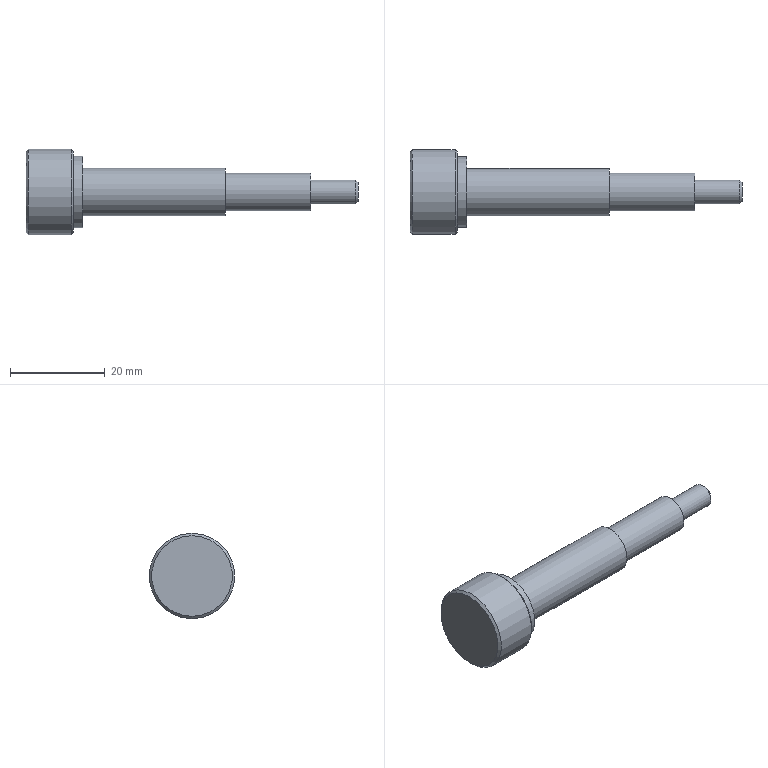Component | NX | CYLINDER_SHAFT | 1 solid | 14 faces | box 70 x 18 x 18 mm | volume 6340 mm3 | plane 6 | cylinder 5 | cone 3 | commonest cylinder face diameters 18 x1 15 x1 10 x1 8 x1 5 x1
STEP:
#1=CARTESIAN_POINT('',(0.,0.,0.));
#2=DIRECTION('',(0.,0.,1.));
#3=DIRECTION('',(1.,0.,0.));
#4=AXIS2_PLACEMENT_3D('',#1,#2,#3);
#5=CARTESIAN_POINT('',(-36.,0.,23.5));
#6=VERTEX_POINT('',#5);
#7=CARTESIAN_POINT('',(-36.,0.,32.));
#8=DIRECTION('',(1.,0.,0.));
#9=DIRECTION('',(0.,0.,-1.));
#10=AXIS2_PLACEMENT_3D('',#7,#8,#9);
#11=CIRCLE('',#10,8.5);
#12=CARTESIAN_POINT('',(-36.,0.,32.));
#13=DIRECTION('',(1.,0.,0.));
#14=DIRECTION('',(0.,0.,-1.));
#15=AXIS2_PLACEMENT_3D('',#12,#13,#14);
#16=PLANE('',#15);
#17=CARTESIAN_POINT('',(0.,0.));
#18=DIRECTION('',(1.,0.));
#19=AXIS2_PLACEMENT_2D('',#17,#18);
#20=CIRCLE('',#19,8.5);
#21=(GEOMETRIC_REPRESENTATION_CONTEXT(2)PARAMETRIC_REPRESENTATION_CONTEXT()REPRESENTATION_CONTEXT('',''));
#22=DEFINITIONAL_REPRESENTATION('',(#20),#21);
#23=PCURVE('',#16,#22);
#24=CARTESIAN_POINT('',(-36.5,0.,32.));
#25=DIRECTION('',(-1.,0.,0.));
#26=DIRECTION('',(0.,0.,1.));
#27=AXIS2_PLACEMENT_3D('',#24,#25,#26);
#28=CONICAL_SURFACE('',#27,9.,0.7854);
#29=CARTESIAN_POINT('',(9.425,-0.5));
#30=DIRECTION('',(-1.,0.));
#31=VECTOR('',#30,1.);
#32=LINE('',#29,#31);
#33=(GEOMETRIC_REPRESENTATION_CONTEXT(2)PARAMETRIC_REPRESENTATION_CONTEXT()REPRESENTATION_CONTEXT('',''));
#34=DEFINITIONAL_REPRESENTATION('',(#32),#33);
#35=PCURVE('',#28,#34);
#36=SURFACE_CURVE('',#11,(#23,#35),.PCURVE_S1.);
#37=EDGE_CURVE('',#6,#6,#36,.T.);
#38=ORIENTED_EDGE('',*,*,#37,.T.);
#39=EDGE_LOOP('',(#38));
#40=FACE_BOUND('',#39,.T.);
#41=CARTESIAN_POINT('',(-36.,0.,24.5));
#42=VERTEX_POINT('',#41);
#43=CARTESIAN_POINT('',(-36.,0.,32.));
#44=DIRECTION('',(1.,0.,0.));
#45=DIRECTION('',(0.,0.,-1.));
#46=AXIS2_PLACEMENT_3D('',#43,#44,#45);
#47=CIRCLE('',#46,7.5);
#48=CARTESIAN_POINT('',(0.,0.));
#49=DIRECTION('',(1.,0.));
#50=AXIS2_PLACEMENT_2D('',#48,#49);
#51=CIRCLE('',#50,7.5);
#52=(GEOMETRIC_REPRESENTATION_CONTEXT(2)PARAMETRIC_REPRESENTATION_CONTEXT()REPRESENTATION_CONTEXT('',''));
#53=DEFINITIONAL_REPRESENTATION('',(#51),#52);
#54=PCURVE('',#16,#53);
#55=CARTESIAN_POINT('',(-36.,0.,32.));
#56=DIRECTION('',(1.,0.,0.));
#57=DIRECTION('',(0.,0.,-1.));
#58=AXIS2_PLACEMENT_3D('',#55,#56,#57);
#59=CYLINDRICAL_SURFACE('',#58,7.5);
#60=CARTESIAN_POINT('',(0.,0.));
#61=DIRECTION('',(1.,0.));
#62=VECTOR('',#61,1.);
#63=LINE('',#60,#62);
#64=(GEOMETRIC_REPRESENTATION_CONTEXT(2)PARAMETRIC_REPRESENTATION_CONTEXT()REPRESENTATION_CONTEXT('',''));
#65=DEFINITIONAL_REPRESENTATION('',(#63),#64);
#66=PCURVE('',#59,#65);
#67=SURFACE_CURVE('',#47,(#54,#66),.PCURVE_S1.);
#68=EDGE_CURVE('',#42,#42,#67,.T.);
#69=ORIENTED_EDGE('',*,*,#68,.F.);
#70=EDGE_LOOP('',(#69));
#71=FACE_BOUND('',#70,.T.);
#72=ADVANCED_FACE('',(#40,#71),#16,.T.);
#73=CARTESIAN_POINT('',(-46.,0.,40.5));
#74=VERTEX_POINT('',#73);
#75=CARTESIAN_POINT('',(-46.,0.,32.));
#76=DIRECTION('',(-1.,0.,0.));
#77=DIRECTION('',(0.,0.,1.));
#78=AXIS2_PLACEMENT_3D('',#75,#76,#77);
#79=CIRCLE('',#78,8.5);
#80=CARTESIAN_POINT('',(-46.,0.,32.));
#81=DIRECTION('',(-1.,0.,0.));
#82=DIRECTION('',(0.,0.,1.));
#83=AXIS2_PLACEMENT_3D('',#80,#81,#82);
#84=PLANE('',#83);
#85=CARTESIAN_POINT('',(0.,0.));
#86=DIRECTION('',(1.,0.));
#87=AXIS2_PLACEMENT_2D('',#85,#86);
#88=CIRCLE('',#87,8.5);
#89=(GEOMETRIC_REPRESENTATION_CONTEXT(2)PARAMETRIC_REPRESENTATION_CONTEXT()REPRESENTATION_CONTEXT('',''));
#90=DEFINITIONAL_REPRESENTATION('',(#88),#89);
#91=PCURVE('',#84,#90);
#92=CARTESIAN_POINT('',(-45.5,0.,32.));
#93=DIRECTION('',(1.,0.,0.));
#94=DIRECTION('',(0.,0.,-1.));
#95=AXIS2_PLACEMENT_3D('',#92,#93,#94);
#96=CONICAL_SURFACE('',#95,9.,0.7854);
#97=CARTESIAN_POINT('',(9.425,-0.5));
#98=DIRECTION('',(-1.,0.));
#99=VECTOR('',#98,1.);
#100=LINE('',#97,#99);
#101=(GEOMETRIC_REPRESENTATION_CONTEXT(2)PARAMETRIC_REPRESENTATION_CONTEXT()REPRESENTATION_CONTEXT('',''));
#102=DEFINITIONAL_REPRESENTATION('',(#100),#101);
#103=PCURVE('',#96,#102);
#104=SURFACE_CURVE('',#79,(#91,#103),.PCURVE_S1.);
#105=EDGE_CURVE('',#74,#74,#104,.T.);
#106=ORIENTED_EDGE('',*,*,#105,.T.);
#107=EDGE_LOOP('',(#106));
#108=FACE_BOUND('',#107,.T.);
#109=ADVANCED_FACE('',(#108),#84,.T.);
#110=CARTESIAN_POINT('',(-45.5,0.,41.));
#111=VERTEX_POINT('',#110);
#112=CARTESIAN_POINT('',(-45.5,-0.,23.));
#113=VERTEX_POINT('',#112);
#114=CARTESIAN_POINT('',(-45.5,0.,32.));
#115=DIRECTION('',(1.,0.,0.));
#116=DIRECTION('',(0.,0.,1.));
#117=AXIS2_PLACEMENT_3D('',#114,#115,#116);
#118=CIRCLE('',#117,9.);
#119=CARTESIAN_POINT('',(-46.,0.,32.));
#120=DIRECTION('',(1.,0.,0.));
#121=DIRECTION('',(0.,0.,-1.));
#122=AXIS2_PLACEMENT_3D('',#119,#120,#121);
#123=CYLINDRICAL_SURFACE('',#122,9.);
#124=CARTESIAN_POINT('',(3.142,0.5));
#125=DIRECTION('',(1.,0.));
#126=VECTOR('',#125,1.);
#127=LINE('',#124,#126);
#128=(GEOMETRIC_REPRESENTATION_CONTEXT(2)PARAMETRIC_REPRESENTATION_CONTEXT()REPRESENTATION_CONTEXT('',''));
#129=DEFINITIONAL_REPRESENTATION('',(#127),#128);
#130=PCURVE('',#123,#129);
#131=CARTESIAN_POINT('',(3.142,0.));
#132=DIRECTION('',(1.,0.));
#133=VECTOR('',#132,1.);
#134=LINE('',#131,#133);
#135=(GEOMETRIC_REPRESENTATION_CONTEXT(2)PARAMETRIC_REPRESENTATION_CONTEXT()REPRESENTATION_CONTEXT('',''));
#136=DEFINITIONAL_REPRESENTATION('',(#134),#135);
#137=PCURVE('',#96,#136);
#138=SURFACE_CURVE('',#118,(#130,#137),.PCURVE_S1.);
#139=EDGE_CURVE('',#111,#113,#138,.T.);
#140=ORIENTED_EDGE('',*,*,#139,.T.);
#141=CARTESIAN_POINT('',(-36.5,0.,23.));
#142=VERTEX_POINT('',#141);
#143=CARTESIAN_POINT('',(-45.5,0.,23.));
#144=CARTESIAN_POINT('',(-36.5,0.,23.));
#145=B_SPLINE_CURVE_WITH_KNOTS('',1,(#143,#144),.UNSPECIFIED.,.F.,.F.,(2,2),(0.5,9.5),.PIECEWISE_BEZIER_KNOTS.);
#146=CARTESIAN_POINT('',(6.283,0.));
#147=DIRECTION('',(0.,1.));
#148=VECTOR('',#147,1.);
#149=LINE('',#146,#148);
#150=(GEOMETRIC_REPRESENTATION_CONTEXT(2)PARAMETRIC_REPRESENTATION_CONTEXT()REPRESENTATION_CONTEXT('',''));
#151=DEFINITIONAL_REPRESENTATION('',(#149),#150);
#152=PCURVE('',#123,#151);
#153=CARTESIAN_POINT('',(0.,0.));
#154=DIRECTION('',(0.,1.));
#155=VECTOR('',#154,1.);
#156=LINE('',#153,#155);
#157=(GEOMETRIC_REPRESENTATION_CONTEXT(2)PARAMETRIC_REPRESENTATION_CONTEXT()REPRESENTATION_CONTEXT('',''));
#158=DEFINITIONAL_REPRESENTATION('',(#156),#157);
#159=PCURVE('',#123,#158);
#160=SEAM_CURVE('',#145,(#152,#159),.PCURVE_S1.);
#161=EDGE_CURVE('',#113,#142,#160,.T.);
#162=ORIENTED_EDGE('',*,*,#161,.T.);
#163=CARTESIAN_POINT('',(-36.5,0.,32.));
#164=DIRECTION('',(-1.,0.,0.));
#165=DIRECTION('',(0.,0.,-1.));
#166=AXIS2_PLACEMENT_3D('',#163,#164,#165);
#167=CIRCLE('',#166,9.);
#168=CARTESIAN_POINT('',(6.283,9.5));
#169=DIRECTION('',(-1.,0.));
#170=VECTOR('',#169,1.);
#171=LINE('',#168,#170);
#172=(GEOMETRIC_REPRESENTATION_CONTEXT(2)PARAMETRIC_REPRESENTATION_CONTEXT()REPRESENTATION_CONTEXT('',''));
#173=DEFINITIONAL_REPRESENTATION('',(#171),#172);
#174=PCURVE('',#123,#173);
#175=CARTESIAN_POINT('',(3.142,0.));
#176=DIRECTION('',(1.,0.));
#177=VECTOR('',#176,1.);
#178=LINE('',#175,#177);
#179=(GEOMETRIC_REPRESENTATION_CONTEXT(2)PARAMETRIC_REPRESENTATION_CONTEXT()REPRESENTATION_CONTEXT('',''));
#180=DEFINITIONAL_REPRESENTATION('',(#178),#179);
#181=PCURVE('',#28,#180);
#182=SURFACE_CURVE('',#167,(#174,#181),.PCURVE_S1.);
#183=EDGE_CURVE('',#142,#142,#182,.T.);
#184=ORIENTED_EDGE('',*,*,#183,.T.);
#185=ORIENTED_EDGE('',*,*,#161,.F.);
#186=CARTESIAN_POINT('',(-45.5,0.,32.));
#187=DIRECTION('',(1.,0.,0.));
#188=DIRECTION('',(0.,0.,1.));
#189=AXIS2_PLACEMENT_3D('',#186,#187,#188);
#190=CIRCLE('',#189,9.);
#191=CARTESIAN_POINT('',(-3.142,0.5));
#192=DIRECTION('',(1.,0.));
#193=VECTOR('',#192,1.);
#194=LINE('',#191,#193);
#195=(GEOMETRIC_REPRESENTATION_CONTEXT(2)PARAMETRIC_REPRESENTATION_CONTEXT()REPRESENTATION_CONTEXT('',''));
#196=DEFINITIONAL_REPRESENTATION('',(#194),#195);
#197=PCURVE('',#123,#196);
#198=CARTESIAN_POINT('',(3.142,0.));
#199=DIRECTION('',(1.,0.));
#200=VECTOR('',#199,1.);
#201=LINE('',#198,#200);
#202=(GEOMETRIC_REPRESENTATION_CONTEXT(2)PARAMETRIC_REPRESENTATION_CONTEXT()REPRESENTATION_CONTEXT('',''));
#203=DEFINITIONAL_REPRESENTATION('',(#201),#202);
#204=PCURVE('',#96,#203);
#205=SURFACE_CURVE('',#190,(#197,#204),.PCURVE_S1.);
#206=EDGE_CURVE('',#113,#111,#205,.T.);
#207=ORIENTED_EDGE('',*,*,#206,.T.);
#208=EDGE_LOOP('',(#140,#162,#184,#185,#207));
#209=FACE_BOUND('',#208,.T.);
#210=ADVANCED_FACE('',(#209),#123,.T.);
#211=CARTESIAN_POINT('',(-34.,0.,27.));
#212=VERTEX_POINT('',#211);
#213=CARTESIAN_POINT('',(-34.,0.,32.));
#214=DIRECTION('',(1.,0.,0.));
#215=DIRECTION('',(0.,0.,-1.));
#216=AXIS2_PLACEMENT_3D('',#213,#214,#215);
#217=CIRCLE('',#216,5.);
#218=CARTESIAN_POINT('',(-34.,0.,32.));
#219=DIRECTION('',(1.,0.,0.));
#220=DIRECTION('',(0.,0.,-1.));
#221=AXIS2_PLACEMENT_3D('',#218,#219,#220);
#222=PLANE('',#221);
#223=CARTESIAN_POINT('',(0.,0.));
#224=DIRECTION('',(1.,0.));
#225=AXIS2_PLACEMENT_2D('',#223,#224);
#226=CIRCLE('',#225,5.);
#227=(GEOMETRIC_REPRESENTATION_CONTEXT(2)PARAMETRIC_REPRESENTATION_CONTEXT()REPRESENTATION_CONTEXT('',''));
#228=DEFINITIONAL_REPRESENTATION('',(#226),#227);
#229=PCURVE('',#222,#228);
#230=CARTESIAN_POINT('',(-34.,0.,32.));
#231=DIRECTION('',(1.,0.,0.));
#232=DIRECTION('',(0.,0.,-1.));
#233=AXIS2_PLACEMENT_3D('',#230,#231,#232);
#234=CYLINDRICAL_SURFACE('',#233,5.);
#235=CARTESIAN_POINT('',(0.,0.));
#236=DIRECTION('',(1.,0.));
#237=VECTOR('',#236,1.);
#238=LINE('',#235,#237);
#239=(GEOMETRIC_REPRESENTATION_CONTEXT(2)PARAMETRIC_REPRESENTATION_CONTEXT()REPRESENTATION_CONTEXT('',''));
#240=DEFINITIONAL_REPRESENTATION('',(#238),#239);
#241=PCURVE('',#234,#240);
#242=SURFACE_CURVE('',#217,(#229,#241),.PCURVE_S1.);
#243=EDGE_CURVE('',#212,#212,#242,.T.);
#244=ORIENTED_EDGE('',*,*,#243,.F.);
#245=EDGE_LOOP('',(#244));
#246=FACE_BOUND('',#245,.T.);
#247=CARTESIAN_POINT('',(-34.,0.,24.5));
#248=VERTEX_POINT('',#247);
#249=CARTESIAN_POINT('',(-34.,0.,32.));
#250=DIRECTION('',(-1.,0.,0.));
#251=DIRECTION('',(0.,0.,-1.));
#252=AXIS2_PLACEMENT_3D('',#249,#250,#251);
#253=CIRCLE('',#252,7.5);
#254=CARTESIAN_POINT('',(7.5,0.));
#255=CARTESIAN_POINT('',(7.5,-12.99));
#256=CARTESIAN_POINT('',(-3.75,-6.495));
#257=CARTESIAN_POINT('',(-15.,-0.));
#258=CARTESIAN_POINT('',(-3.75,6.495));
#259=CARTESIAN_POINT('',(7.5,12.99));
#260=CARTESIAN_POINT('',(7.5,0.));
#261=(BOUNDED_CURVE()B_SPLINE_CURVE(2,(#254,#255,#256,#257,#258,#259,#260),.UNSPECIFIED.,.T.,.F.)B_SPLINE_CURVE_WITH_KNOTS((1,2,2,2,2,1),(-2.094,0.,2.094,4.189,6.283,8.378),.UNSPECIFIED.)CURVE()GEOMETRIC_REPRESENTATION_ITEM()RATIONAL_B_SPLINE_CURVE((1.,0.5,1.,0.5,1.,0.5,1.))REPRESENTATION_ITEM(''));
#262=(GEOMETRIC_REPRESENTATION_CONTEXT(2)PARAMETRIC_REPRESENTATION_CONTEXT()REPRESENTATION_CONTEXT('',''));
#263=DEFINITIONAL_REPRESENTATION('',(#261),#262);
#264=PCURVE('',#222,#263);
#265=CARTESIAN_POINT('',(6.283,2.));
#266=DIRECTION('',(-1.,0.));
#267=VECTOR('',#266,1.);
#268=LINE('',#265,#267);
#269=(GEOMETRIC_REPRESENTATION_CONTEXT(2)PARAMETRIC_REPRESENTATION_CONTEXT()REPRESENTATION_CONTEXT('',''));
#270=DEFINITIONAL_REPRESENTATION('',(#268),#269);
#271=PCURVE('',#59,#270);
#272=SURFACE_CURVE('',#253,(#264,#271),.PCURVE_S1.);
#273=EDGE_CURVE('',#248,#248,#272,.T.);
#274=ORIENTED_EDGE('',*,*,#273,.F.);
#275=EDGE_LOOP('',(#274));
#276=FACE_BOUND('',#275,.T.);
#277=ADVANCED_FACE('',(#246,#276),#222,.T.);
#278=ORIENTED_EDGE('',*,*,#273,.T.);
#279=CARTESIAN_POINT('',(-36.,-0.,24.5));
#280=CARTESIAN_POINT('',(-34.,-0.,24.5));
#281=B_SPLINE_CURVE_WITH_KNOTS('',1,(#279,#280),.UNSPECIFIED.,.F.,.F.,(2,2),(0.,2.),.PIECEWISE_BEZIER_KNOTS.);
#282=CARTESIAN_POINT('',(0.,0.));
#283=DIRECTION('',(0.,1.));
#284=VECTOR('',#283,1.);
#285=LINE('',#282,#284);
#286=(GEOMETRIC_REPRESENTATION_CONTEXT(2)PARAMETRIC_REPRESENTATION_CONTEXT()REPRESENTATION_CONTEXT('',''));
#287=DEFINITIONAL_REPRESENTATION('',(#285),#286);
#288=PCURVE('',#59,#287);
#289=CARTESIAN_POINT('',(6.283,0.));
#290=DIRECTION('',(0.,1.));
#291=VECTOR('',#290,1.);
#292=LINE('',#289,#291);
#293=(GEOMETRIC_REPRESENTATION_CONTEXT(2)PARAMETRIC_REPRESENTATION_CONTEXT()REPRESENTATION_CONTEXT('',''));
#294=DEFINITIONAL_REPRESENTATION('',(#292),#293);
#295=PCURVE('',#59,#294);
#296=SEAM_CURVE('',#281,(#288,#295),.PCURVE_S1.);
#297=EDGE_CURVE('',#42,#248,#296,.T.);
#298=ORIENTED_EDGE('',*,*,#297,.F.);
#299=ORIENTED_EDGE('',*,*,#68,.T.);
#300=ORIENTED_EDGE('',*,*,#297,.T.);
#301=EDGE_LOOP('',(#278,#298,#299,#300));
#302=FACE_BOUND('',#301,.T.);
#303=ADVANCED_FACE('',(#302),#59,.T.);
#304=CARTESIAN_POINT('',(-4.,0.,28.));
#305=VERTEX_POINT('',#304);
#306=CARTESIAN_POINT('',(-4.,0.,32.));
#307=DIRECTION('',(1.,0.,0.));
#308=DIRECTION('',(0.,0.,-1.));
#309=AXIS2_PLACEMENT_3D('',#306,#307,#308);
#310=CIRCLE('',#309,4.);
#311=CARTESIAN_POINT('',(-4.,0.,32.));
#312=DIRECTION('',(1.,0.,0.));
#313=DIRECTION('',(0.,0.,-1.));
#314=AXIS2_PLACEMENT_3D('',#311,#312,#313);
#315=PLANE('',#314);
#316=CARTESIAN_POINT('',(0.,0.));
#317=DIRECTION('',(1.,0.));
#318=AXIS2_PLACEMENT_2D('',#316,#317);
#319=CIRCLE('',#318,4.);
#320=(GEOMETRIC_REPRESENTATION_CONTEXT(2)PARAMETRIC_REPRESENTATION_CONTEXT()REPRESENTATION_CONTEXT('',''));
#321=DEFINITIONAL_REPRESENTATION('',(#319),#320);
#322=PCURVE('',#315,#321);
#323=CARTESIAN_POINT('',(-4.,0.,32.));
#324=DIRECTION('',(1.,0.,0.));
#325=DIRECTION('',(0.,0.,-1.));
#326=AXIS2_PLACEMENT_3D('',#323,#324,#325);
#327=CYLINDRICAL_SURFACE('',#326,4.);
#328=CARTESIAN_POINT('',(0.,0.));
#329=DIRECTION('',(1.,0.));
#330=VECTOR('',#329,1.);
#331=LINE('',#328,#330);
#332=(GEOMETRIC_REPRESENTATION_CONTEXT(2)PARAMETRIC_REPRESENTATION_CONTEXT()REPRESENTATION_CONTEXT('',''));
#333=DEFINITIONAL_REPRESENTATION('',(#331),#332);
#334=PCURVE('',#327,#333);
#335=SURFACE_CURVE('',#310,(#322,#334),.PCURVE_S1.);
#336=EDGE_CURVE('',#305,#305,#335,.T.);
#337=ORIENTED_EDGE('',*,*,#336,.F.);
#338=EDGE_LOOP('',(#337));
#339=FACE_BOUND('',#338,.T.);
#340=CARTESIAN_POINT('',(-4.,0.,27.));
#341=VERTEX_POINT('',#340);
#342=CARTESIAN_POINT('',(-4.,0.,32.));
#343=DIRECTION('',(-1.,0.,0.));
#344=DIRECTION('',(0.,0.,-1.));
#345=AXIS2_PLACEMENT_3D('',#342,#343,#344);
#346=CIRCLE('',#345,5.);
#347=CARTESIAN_POINT('',(5.,0.));
#348=CARTESIAN_POINT('',(5.,-8.66));
#349=CARTESIAN_POINT('',(-2.5,-4.33));
#350=CARTESIAN_POINT('',(-10.,-0.));
#351=CARTESIAN_POINT('',(-2.5,4.33));
#352=CARTESIAN_POINT('',(5.,8.66));
#353=CARTESIAN_POINT('',(5.,0.));
#354=(BOUNDED_CURVE()B_SPLINE_CURVE(2,(#347,#348,#349,#350,#351,#352,#353),.UNSPECIFIED.,.T.,.F.)B_SPLINE_CURVE_WITH_KNOTS((1,2,2,2,2,1),(-2.094,0.,2.094,4.189,6.283,8.378),.UNSPECIFIED.)CURVE()GEOMETRIC_REPRESENTATION_ITEM()RATIONAL_B_SPLINE_CURVE((1.,0.5,1.,0.5,1.,0.5,1.))REPRESENTATION_ITEM(''));
#355=(GEOMETRIC_REPRESENTATION_CONTEXT(2)PARAMETRIC_REPRESENTATION_CONTEXT()REPRESENTATION_CONTEXT('',''));
#356=DEFINITIONAL_REPRESENTATION('',(#354),#355);
#357=PCURVE('',#315,#356);
#358=CARTESIAN_POINT('',(6.283,30.));
#359=DIRECTION('',(-1.,0.));
#360=VECTOR('',#359,1.);
#361=LINE('',#358,#360);
#362=(GEOMETRIC_REPRESENTATION_CONTEXT(2)PARAMETRIC_REPRESENTATION_CONTEXT()REPRESENTATION_CONTEXT('',''));
#363=DEFINITIONAL_REPRESENTATION('',(#361),#362);
#364=PCURVE('',#234,#363);
#365=SURFACE_CURVE('',#346,(#357,#364),.PCURVE_S1.);
#366=EDGE_CURVE('',#341,#341,#365,.T.);
#367=ORIENTED_EDGE('',*,*,#366,.F.);
#368=EDGE_LOOP('',(#367));
#369=FACE_BOUND('',#368,.T.);
#370=ADVANCED_FACE('',(#339,#369),#315,.T.);
#371=ORIENTED_EDGE('',*,*,#366,.T.);
#372=CARTESIAN_POINT('',(-34.,-0.,27.));
#373=CARTESIAN_POINT('',(-4.,-0.,27.));
#374=B_SPLINE_CURVE_WITH_KNOTS('',1,(#372,#373),.UNSPECIFIED.,.F.,.F.,(2,2),(0.,30.),.PIECEWISE_BEZIER_KNOTS.);
#375=CARTESIAN_POINT('',(0.,0.));
#376=DIRECTION('',(0.,1.));
#377=VECTOR('',#376,1.);
#378=LINE('',#375,#377);
#379=(GEOMETRIC_REPRESENTATION_CONTEXT(2)PARAMETRIC_REPRESENTATION_CONTEXT()REPRESENTATION_CONTEXT('',''));
#380=DEFINITIONAL_REPRESENTATION('',(#378),#379);
#381=PCURVE('',#234,#380);
#382=CARTESIAN_POINT('',(6.283,0.));
#383=DIRECTION('',(0.,1.));
#384=VECTOR('',#383,1.);
#385=LINE('',#382,#384);
#386=(GEOMETRIC_REPRESENTATION_CONTEXT(2)PARAMETRIC_REPRESENTATION_CONTEXT()REPRESENTATION_CONTEXT('',''));
#387=DEFINITIONAL_REPRESENTATION('',(#385),#386);
#388=PCURVE('',#234,#387);
#389=SEAM_CURVE('',#374,(#381,#388),.PCURVE_S1.);
#390=EDGE_CURVE('',#212,#341,#389,.T.);
#391=ORIENTED_EDGE('',*,*,#390,.F.);
#392=ORIENTED_EDGE('',*,*,#243,.T.);
#393=ORIENTED_EDGE('',*,*,#390,.T.);
#394=EDGE_LOOP('',(#371,#391,#392,#393));
#395=FACE_BOUND('',#394,.T.);
#396=ADVANCED_FACE('',(#395),#234,.T.);
#397=CARTESIAN_POINT('',(14.,0.,29.5));
#398=VERTEX_POINT('',#397);
#399=CARTESIAN_POINT('',(14.,0.,32.));
#400=DIRECTION('',(1.,0.,0.));
#401=DIRECTION('',(0.,0.,-1.));
#402=AXIS2_PLACEMENT_3D('',#399,#400,#401);
#403=CIRCLE('',#402,2.5);
#404=CARTESIAN_POINT('',(14.,0.,32.));
#405=DIRECTION('',(1.,0.,0.));
#406=DIRECTION('',(0.,0.,-1.));
#407=AXIS2_PLACEMENT_3D('',#404,#405,#406);
#408=PLANE('',#407);
#409=CARTESIAN_POINT('',(0.,0.));
#410=DIRECTION('',(1.,0.));
#411=AXIS2_PLACEMENT_2D('',#409,#410);
#412=CIRCLE('',#411,2.5);
#413=(GEOMETRIC_REPRESENTATION_CONTEXT(2)PARAMETRIC_REPRESENTATION_CONTEXT()REPRESENTATION_CONTEXT('',''));
#414=DEFINITIONAL_REPRESENTATION('',(#412),#413);
#415=PCURVE('',#408,#414);
#416=CARTESIAN_POINT('',(14.,0.,32.));
#417=DIRECTION('',(1.,0.,0.));
#418=DIRECTION('',(0.,0.,-1.));
#419=AXIS2_PLACEMENT_3D('',#416,#417,#418);
#420=CYLINDRICAL_SURFACE('',#419,2.5);
#421=CARTESIAN_POINT('',(0.,0.));
#422=DIRECTION('',(1.,0.));
#423=VECTOR('',#422,1.);
#424=LINE('',#421,#423);
#425=(GEOMETRIC_REPRESENTATION_CONTEXT(2)PARAMETRIC_REPRESENTATION_CONTEXT()REPRESENTATION_CONTEXT('',''));
#426=DEFINITIONAL_REPRESENTATION('',(#424),#425);
#427=PCURVE('',#420,#426);
#428=SURFACE_CURVE('',#403,(#415,#427),.PCURVE_S1.);
#429=EDGE_CURVE('',#398,#398,#428,.T.);
#430=ORIENTED_EDGE('',*,*,#429,.F.);
#431=EDGE_LOOP('',(#430));
#432=FACE_BOUND('',#431,.T.);
#433=CARTESIAN_POINT('',(14.,0.,28.));
#434=VERTEX_POINT('',#433);
#435=CARTESIAN_POINT('',(14.,0.,32.));
#436=DIRECTION('',(-1.,0.,0.));
#437=DIRECTION('',(0.,0.,-1.));
#438=AXIS2_PLACEMENT_3D('',#435,#436,#437);
#439=CIRCLE('',#438,4.);
#440=CARTESIAN_POINT('',(4.,0.));
#441=CARTESIAN_POINT('',(4.,-6.928));
#442=CARTESIAN_POINT('',(-2.,-3.464));
#443=CARTESIAN_POINT('',(-8.,-0.));
#444=CARTESIAN_POINT('',(-2.,3.464));
#445=CARTESIAN_POINT('',(4.,6.928));
#446=CARTESIAN_POINT('',(4.,0.));
#447=(BOUNDED_CURVE()B_SPLINE_CURVE(2,(#440,#441,#442,#443,#444,#445,#446),.UNSPECIFIED.,.T.,.F.)B_SPLINE_CURVE_WITH_KNOTS((1,2,2,2,2,1),(-2.094,0.,2.094,4.189,6.283,8.378),.UNSPECIFIED.)CURVE()GEOMETRIC_REPRESENTATION_ITEM()RATIONAL_B_SPLINE_CURVE((1.,0.5,1.,0.5,1.,0.5,1.))REPRESENTATION_ITEM(''));
#448=(GEOMETRIC_REPRESENTATION_CONTEXT(2)PARAMETRIC_REPRESENTATION_CONTEXT()REPRESENTATION_CONTEXT('',''));
#449=DEFINITIONAL_REPRESENTATION('',(#447),#448);
#450=PCURVE('',#408,#449);
#451=CARTESIAN_POINT('',(6.283,18.));
#452=DIRECTION('',(-1.,0.));
#453=VECTOR('',#452,1.);
#454=LINE('',#451,#453);
#455=(GEOMETRIC_REPRESENTATION_CONTEXT(2)PARAMETRIC_REPRESENTATION_CONTEXT()REPRESENTATION_CONTEXT('',''));
#456=DEFINITIONAL_REPRESENTATION('',(#454),#455);
#457=PCURVE('',#327,#456);
#458=SURFACE_CURVE('',#439,(#450,#457),.PCURVE_S1.);
#459=EDGE_CURVE('',#434,#434,#458,.T.);
#460=ORIENTED_EDGE('',*,*,#459,.F.);
#461=EDGE_LOOP('',(#460));
#462=FACE_BOUND('',#461,.T.);
#463=ADVANCED_FACE('',(#432,#462),#408,.T.);
#464=ORIENTED_EDGE('',*,*,#459,.T.);
#465=CARTESIAN_POINT('',(-4.,-0.,28.));
#466=CARTESIAN_POINT('',(14.,-0.,28.));
#467=B_SPLINE_CURVE_WITH_KNOTS('',1,(#465,#466),.UNSPECIFIED.,.F.,.F.,(2,2),(0.,18.),.PIECEWISE_BEZIER_KNOTS.);
#468=CARTESIAN_POINT('',(0.,0.));
#469=DIRECTION('',(0.,1.));
#470=VECTOR('',#469,1.);
#471=LINE('',#468,#470);
#472=(GEOMETRIC_REPRESENTATION_CONTEXT(2)PARAMETRIC_REPRESENTATION_CONTEXT()REPRESENTATION_CONTEXT('',''));
#473=DEFINITIONAL_REPRESENTATION('',(#471),#472);
#474=PCURVE('',#327,#473);
#475=CARTESIAN_POINT('',(6.283,0.));
#476=DIRECTION('',(0.,1.));
#477=VECTOR('',#476,1.);
#478=LINE('',#475,#477);
#479=(GEOMETRIC_REPRESENTATION_CONTEXT(2)PARAMETRIC_REPRESENTATION_CONTEXT()REPRESENTATION_CONTEXT('',''));
#480=DEFINITIONAL_REPRESENTATION('',(#478),#479);
#481=PCURVE('',#327,#480);
#482=SEAM_CURVE('',#467,(#474,#481),.PCURVE_S1.);
#483=EDGE_CURVE('',#305,#434,#482,.T.);
#484=ORIENTED_EDGE('',*,*,#483,.F.);
#485=ORIENTED_EDGE('',*,*,#336,.T.);
#486=ORIENTED_EDGE('',*,*,#483,.T.);
#487=EDGE_LOOP('',(#464,#484,#485,#486));
#488=FACE_BOUND('',#487,.T.);
#489=ADVANCED_FACE('',(#488),#327,.T.);
#490=CARTESIAN_POINT('',(24.,0.,30.));
#491=VERTEX_POINT('',#490);
#492=CARTESIAN_POINT('',(24.,0.,32.));
#493=DIRECTION('',(1.,0.,0.));
#494=DIRECTION('',(0.,0.,-1.));
#495=AXIS2_PLACEMENT_3D('',#492,#493,#494);
#496=CIRCLE('',#495,2.);
#497=CARTESIAN_POINT('',(24.,0.,32.));
#498=DIRECTION('',(1.,0.,0.));
#499=DIRECTION('',(0.,0.,-1.));
#500=AXIS2_PLACEMENT_3D('',#497,#498,#499);
#501=PLANE('',#500);
#502=CARTESIAN_POINT('',(0.,0.));
#503=DIRECTION('',(1.,0.));
#504=AXIS2_PLACEMENT_2D('',#502,#503);
#505=CIRCLE('',#504,2.);
#506=(GEOMETRIC_REPRESENTATION_CONTEXT(2)PARAMETRIC_REPRESENTATION_CONTEXT()REPRESENTATION_CONTEXT('',''));
#507=DEFINITIONAL_REPRESENTATION('',(#505),#506);
#508=PCURVE('',#501,#507);
#509=CARTESIAN_POINT('',(23.5,0.,32.));
#510=DIRECTION('',(-1.,0.,0.));
#511=DIRECTION('',(0.,0.,1.));
#512=AXIS2_PLACEMENT_3D('',#509,#510,#511);
#513=CONICAL_SURFACE('',#512,2.5,0.7854);
#514=CARTESIAN_POINT('',(9.425,-0.5));
#515=DIRECTION('',(-1.,0.));
#516=VECTOR('',#515,1.);
#517=LINE('',#514,#516);
#518=(GEOMETRIC_REPRESENTATION_CONTEXT(2)PARAMETRIC_REPRESENTATION_CONTEXT()REPRESENTATION_CONTEXT('',''));
#519=DEFINITIONAL_REPRESENTATION('',(#517),#518);
#520=PCURVE('',#513,#519);
#521=SURFACE_CURVE('',#496,(#508,#520),.PCURVE_S1.);
#522=EDGE_CURVE('',#491,#491,#521,.T.);
#523=ORIENTED_EDGE('',*,*,#522,.T.);
#524=EDGE_LOOP('',(#523));
#525=FACE_BOUND('',#524,.T.);
#526=ADVANCED_FACE('',(#525),#501,.T.);
#527=CARTESIAN_POINT('',(23.5,0.,29.5));
#528=VERTEX_POINT('',#527);
#529=CARTESIAN_POINT('',(23.5,0.,32.));
#530=DIRECTION('',(-1.,0.,0.));
#531=DIRECTION('',(0.,0.,-1.));
#532=AXIS2_PLACEMENT_3D('',#529,#530,#531);
#533=CIRCLE('',#532,2.5);
#534=CARTESIAN_POINT('',(6.283,9.5));
#535=DIRECTION('',(-1.,0.));
#536=VECTOR('',#535,1.);
#537=LINE('',#534,#536);
#538=(GEOMETRIC_REPRESENTATION_CONTEXT(2)PARAMETRIC_REPRESENTATION_CONTEXT()REPRESENTATION_CONTEXT('',''));
#539=DEFINITIONAL_REPRESENTATION('',(#537),#538);
#540=PCURVE('',#420,#539);
#541=CARTESIAN_POINT('',(3.142,0.));
#542=DIRECTION('',(1.,0.));
#543=VECTOR('',#542,1.);
#544=LINE('',#541,#543);
#545=(GEOMETRIC_REPRESENTATION_CONTEXT(2)PARAMETRIC_REPRESENTATION_CONTEXT()REPRESENTATION_CONTEXT('',''));
#546=DEFINITIONAL_REPRESENTATION('',(#544),#545);
#547=PCURVE('',#513,#546);
#548=SURFACE_CURVE('',#533,(#540,#547),.PCURVE_S1.);
#549=EDGE_CURVE('',#528,#528,#548,.T.);
#550=ORIENTED_EDGE('',*,*,#549,.T.);
#551=CARTESIAN_POINT('',(14.,0.,29.5));
#552=CARTESIAN_POINT('',(23.5,0.,29.5));
#553=B_SPLINE_CURVE_WITH_KNOTS('',1,(#551,#552),.UNSPECIFIED.,.F.,.F.,(2,2),(0.,9.5),.PIECEWISE_BEZIER_KNOTS.);
#554=CARTESIAN_POINT('',(0.,0.));
#555=DIRECTION('',(0.,1.));
#556=VECTOR('',#555,1.);
#557=LINE('',#554,#556);
#558=(GEOMETRIC_REPRESENTATION_CONTEXT(2)PARAMETRIC_REPRESENTATION_CONTEXT()REPRESENTATION_CONTEXT('',''));
#559=DEFINITIONAL_REPRESENTATION('',(#557),#558);
#560=PCURVE('',#420,#559);
#561=CARTESIAN_POINT('',(6.283,0.));
#562=DIRECTION('',(0.,1.));
#563=VECTOR('',#562,1.);
#564=LINE('',#561,#563);
#565=(GEOMETRIC_REPRESENTATION_CONTEXT(2)PARAMETRIC_REPRESENTATION_CONTEXT()REPRESENTATION_CONTEXT('',''));
#566=DEFINITIONAL_REPRESENTATION('',(#564),#565);
#567=PCURVE('',#420,#566);
#568=SEAM_CURVE('',#553,(#560,#567),.PCURVE_S1.);
#569=EDGE_CURVE('',#398,#528,#568,.T.);
#570=ORIENTED_EDGE('',*,*,#569,.F.);
#571=ORIENTED_EDGE('',*,*,#429,.T.);
#572=ORIENTED_EDGE('',*,*,#569,.T.);
#573=EDGE_LOOP('',(#550,#570,#571,#572));
#574=FACE_BOUND('',#573,.T.);
#575=ADVANCED_FACE('',(#574),#420,.T.);
#576=ORIENTED_EDGE('',*,*,#522,.F.);
#577=CARTESIAN_POINT('',(24.,0.,30.));
#578=CARTESIAN_POINT('',(23.5,0.,29.5));
#579=B_SPLINE_CURVE_WITH_KNOTS('',1,(#577,#578),.UNSPECIFIED.,.F.,.F.,(2,2),(-0.7071,0.),.PIECEWISE_BEZIER_KNOTS.);
#580=CARTESIAN_POINT('',(9.425,0.));
#581=DIRECTION('',(0.,1.));
#582=VECTOR('',#581,1.);
#583=LINE('',#580,#582);
#584=(GEOMETRIC_REPRESENTATION_CONTEXT(2)PARAMETRIC_REPRESENTATION_CONTEXT()REPRESENTATION_CONTEXT('',''));
#585=DEFINITIONAL_REPRESENTATION('',(#583),#584);
#586=PCURVE('',#513,#585);
#587=CARTESIAN_POINT('',(3.142,0.));
#588=DIRECTION('',(0.,1.));
#589=VECTOR('',#588,1.);
#590=LINE('',#587,#589);
#591=(GEOMETRIC_REPRESENTATION_CONTEXT(2)PARAMETRIC_REPRESENTATION_CONTEXT()REPRESENTATION_CONTEXT('',''));
#592=DEFINITIONAL_REPRESENTATION('',(#590),#591);
#593=PCURVE('',#513,#592);
#594=SEAM_CURVE('',#579,(#586,#593),.PCURVE_S1.);
#595=EDGE_CURVE('',#491,#528,#594,.T.);
#596=ORIENTED_EDGE('',*,*,#595,.T.);
#597=ORIENTED_EDGE('',*,*,#549,.F.);
#598=ORIENTED_EDGE('',*,*,#595,.F.);
#599=EDGE_LOOP('',(#576,#596,#597,#598));
#600=FACE_BOUND('',#599,.T.);
#601=ADVANCED_FACE('',(#600),#513,.T.);
#602=ORIENTED_EDGE('',*,*,#105,.F.);
#603=CARTESIAN_POINT('',(-46.,0.,40.5));
#604=CARTESIAN_POINT('',(-45.5,0.,41.));
#605=B_SPLINE_CURVE_WITH_KNOTS('',1,(#603,#604),.UNSPECIFIED.,.F.,.F.,(2,2),(-0.7071,0.),.PIECEWISE_BEZIER_KNOTS.);
#606=CARTESIAN_POINT('',(9.425,0.));
#607=DIRECTION('',(0.,1.));
#608=VECTOR('',#607,1.);
#609=LINE('',#606,#608);
#610=(GEOMETRIC_REPRESENTATION_CONTEXT(2)PARAMETRIC_REPRESENTATION_CONTEXT()REPRESENTATION_CONTEXT('',''));
#611=DEFINITIONAL_REPRESENTATION('',(#609),#610);
#612=PCURVE('',#96,#611);
#613=CARTESIAN_POINT('',(3.142,0.));
#614=DIRECTION('',(0.,1.));
#615=VECTOR('',#614,1.);
#616=LINE('',#613,#615);
#617=(GEOMETRIC_REPRESENTATION_CONTEXT(2)PARAMETRIC_REPRESENTATION_CONTEXT()REPRESENTATION_CONTEXT('',''));
#618=DEFINITIONAL_REPRESENTATION('',(#616),#617);
#619=PCURVE('',#96,#618);
#620=SEAM_CURVE('',#605,(#612,#619),.PCURVE_S1.);
#621=EDGE_CURVE('',#74,#111,#620,.T.);
#622=ORIENTED_EDGE('',*,*,#621,.T.);
#623=ORIENTED_EDGE('',*,*,#206,.F.);
#624=ORIENTED_EDGE('',*,*,#139,.F.);
#625=ORIENTED_EDGE('',*,*,#621,.F.);
#626=EDGE_LOOP('',(#602,#622,#623,#624,#625));
#627=FACE_BOUND('',#626,.T.);
#628=ADVANCED_FACE('',(#627),#96,.T.);
#629=ORIENTED_EDGE('',*,*,#37,.F.);
#630=CARTESIAN_POINT('',(-36.,0.,23.5));
#631=CARTESIAN_POINT('',(-36.5,0.,23.));
#632=B_SPLINE_CURVE_WITH_KNOTS('',1,(#630,#631),.UNSPECIFIED.,.F.,.F.,(2,2),(-0.7071,0.),.PIECEWISE_BEZIER_KNOTS.);
#633=CARTESIAN_POINT('',(9.425,0.));
#634=DIRECTION('',(0.,1.));
#635=VECTOR('',#634,1.);
#636=LINE('',#633,#635);
#637=(GEOMETRIC_REPRESENTATION_CONTEXT(2)PARAMETRIC_REPRESENTATION_CONTEXT()REPRESENTATION_CONTEXT('',''));
#638=DEFINITIONAL_REPRESENTATION('',(#636),#637);
#639=PCURVE('',#28,#638);
#640=CARTESIAN_POINT('',(3.142,0.));
#641=DIRECTION('',(0.,1.));
#642=VECTOR('',#641,1.);
#643=LINE('',#640,#642);
#644=(GEOMETRIC_REPRESENTATION_CONTEXT(2)PARAMETRIC_REPRESENTATION_CONTEXT()REPRESENTATION_CONTEXT('',''));
#645=DEFINITIONAL_REPRESENTATION('',(#643),#644);
#646=PCURVE('',#28,#645);
#647=SEAM_CURVE('',#632,(#639,#646),.PCURVE_S1.);
#648=EDGE_CURVE('',#6,#142,#647,.T.);
#649=ORIENTED_EDGE('',*,*,#648,.T.);
#650=ORIENTED_EDGE('',*,*,#183,.F.);
#651=ORIENTED_EDGE('',*,*,#648,.F.);
#652=EDGE_LOOP('',(#629,#649,#650,#651));
#653=FACE_BOUND('',#652,.T.);
#654=ADVANCED_FACE('',(#653),#28,.T.);
#655=CLOSED_SHELL('',(#72,#109,#210,#277,#303,#370,#396,#463,#489,#526,#575,#601,#628,#654));
#656=MANIFOLD_SOLID_BREP('',#655);
#657=(LENGTH_UNIT()NAMED_UNIT(*)SI_UNIT(.MILLI.,.METRE.));
#658=UNCERTAINTY_MEASURE_WITH_UNIT(LENGTH_MEASURE(0.00001),#657,'','');
#659=(NAMED_UNIT(*)PLANE_ANGLE_UNIT()SI_UNIT($,.RADIAN.));
#660=(NAMED_UNIT(*)SI_UNIT($,.STERADIAN.)SOLID_ANGLE_UNIT());
#661=(GEOMETRIC_REPRESENTATION_CONTEXT(3)GLOBAL_UNCERTAINTY_ASSIGNED_CONTEXT((#658))GLOBAL_UNIT_ASSIGNED_CONTEXT((#657,#659,#660))REPRESENTATION_CONTEXT('',''));
#662=ADVANCED_BREP_SHAPE_REPRESENTATION('',(#4,#656),#661);